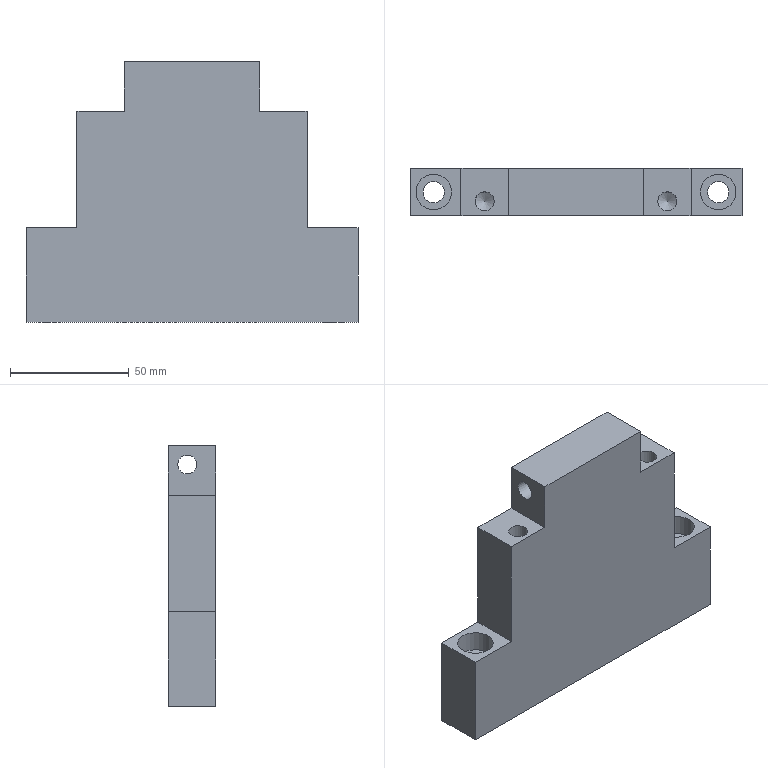Component | NX | BRACKET_2 | 1 solid | 25 faces | volume 219969 mm3 | plane 16 | cylinder 7 | cone 2 | commonest cylinder face diameters 8 x3 9 x2 15 x2